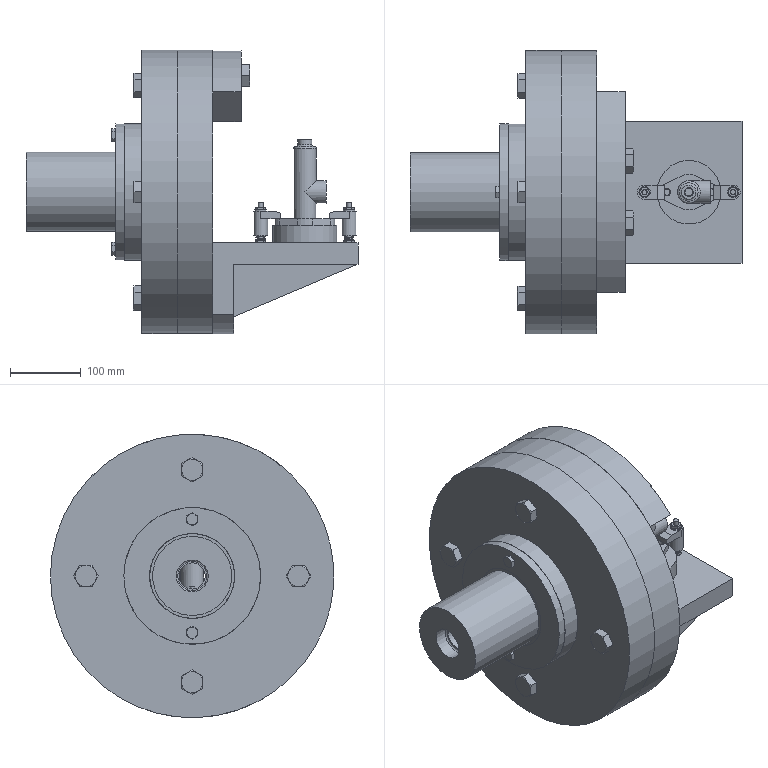Assembly | NX | mm | 33 component files | 33 solids | 523 faces | box 468.52 x 400 x 400 mm | volume 16620251 mm3 | plane 239 | cone 149 | cylinder 110 | torus 15 | spline 10 | commonest cylinder face diameters 19.623 x12 10 x10 6.985 x8 23 x8 27.7 x6 20 x5 9 x4 9.732 x4
Bill of materials:
unnamed part 1 | 1 |  | Solid stepped cylindrical pin: a short large-diameter head and a smaller coaxial shank, with chamfered edges.
unnamed part 2 | 1 |  | Tee-shaped tubular body. A vertical tube has a smaller stepped spigot at the top. A shorter side branch joins it at right angles. A thin two-lobed flange with two holes sits near the bottom, and the tube continues a short way below the flange.
unnamed part 3 | 1 |  | Stepped cylindrical pin with a thin round collar. Above the collar is a head with two parallel flats. Below it are a short undercut neck and a cylindrical shank with chamfered ends.
unnamed part 4 | 1 |  | Flanged bushing. A long cylindrical body leads to a short step, then a large round flange, then a short tapered nose. A central through bore has a counterbore or recessed ring on the flange face, and the flange has two small holes.
unnamed part 5 | 1 |  | Flat arc-shaped plate (annular sector) with radial-cut ends. One arc-shaped slot with rounded ends runs through it, concentric with the plate.
GB-T5782-2000,M20x80 | 6 |  | Hexagon Head Bolt, GB-T 5782-2000,M20x80
GB-T6172_1-2000,M8x1.25 | 4 |  | Hexagon Thin Nut, Chamfered, GB-T 6172.1-2000,M8x1.25
unnamed part 6 | 1 |  | Thick round disc with a central through hole and four small through holes equally spaced on a circle.
unnamed part 7 | 1 |  | Thin flat ring with a large central opening and two small through holes on opposite sides.
GB-T5783-2000,M10x30 | 2 |  | Hex-head bolt-like part: a hexagonal head with chamfered corners, a thin round washer face or collar under the head, and a smooth plain cylindrical shank with a chamfered flat end.
GB-T95-2002,M8 | 2 |  | Plain Washer, GB-T 95-2002,M8
unnamed part 8 | 2 |  | Solid cylinder with a flat lug on top. The lug has one rounded end, which holds a circular hole above the cylinder, and extends sideways to a rectangular end with a sloped top face.
unnamed part 9 | 2 |  | Helical coil spring of round wire with a constant diameter and roughly constant pitch. The end coils look closed and flattened.
GB-T70.1-2000,M12x40 | 2 |  | Hexagon Socket Head Cap Screw, GB-T 70.1-2000,M12x40
GB-T119.1-2000,10x50 | 2 |  | Parallel Pin, GB-T 119.1-2000,10x50
unnamed part 10 | 2 |  | Plain solid cylindrical rod or pin with flat ends.
unnamed part 11 | 1 |  | Thick round disc with a central through hole. It has four holes equally spaced on a circle, a group of three holes near one edge, and a group of five holes near the opposite edge (one larger hole with four smaller holes around it).
unnamed part 12 | 1 |  | Bracket block with a flat rectangular face and a cylindrical boss with a central bore. The block has a wedge-shaped (tapered) side profile with a small square foot at one end. Several small holes are visible, and the views also show four through holes, two slot-like features and a curved edge.
Mates:
1. concentric | adapter_plate 1 edge | faceplate 1 edge
2. concentric | CA614_spindle 1 edge | adapter_plate 1 edge
3. concentric | locking_plate 1 edge | CA614_spindle 1 edge
4. concentric | balance_block 1 edge | faceplate 1 edge
5. concentric | angle_iron 1 edge | faceplate 1 edge
6. concentric | cylinder_body 1 edge | angle_iron 1 edge
7. concentric | B_loc_pin 1 edge | angle_iron 1 edge
8. concentric | fixed_dowel_pin 1 edge | angle_iron 1 edge
9. distance | hook_clamp_plate 2 face | angle_iron 1 face
10. touch align | screw_rod 2 face | hook_clamp_plate 2 face
11. touch align | hook_clamp_plate 2 face | angle_iron 1 face
12. distance | screw_rod 2 face | hook_clamp_plate 2 face
13. concentric | GB-T6172_1-2000_M8x1_25 4 edge | angle_iron 1 arc
14. concentric | spring 2 edge | GB-T6172_1-2000_M8x1_25 4 edge
15. concentric | GB-T95-2002_M8 2 edge | hook_clamp_plate 2 edge
16. concentric | GB-T6172_1-2000_M8x1_25 3 edge | GB-T95-2002_M8 2 edge
17. bond | angle_iron 1 component | assembly component
18. bond | hook_clamp_plate 2 component | assembly component
19. bond | screw_rod 2 component | assembly component
20. bond | GB-T6172_1-2000_M8x1_25 4 component | assembly component
21. bond | spring 2 component | assembly component
22. bond | GB-T6172_1-2000_M8x1_25 3 component | assembly component
23. bond | GB-T95-2002_M8 2 component | assembly component
24. bond | hook_clamp_plate 1 component | assembly component
25. bond | screw_rod 1 component | assembly component
26. bond | GB-T6172_1-2000_M8x1_25 2 component | assembly component
27. bond | spring 1 component | assembly component
28. bond | GB-T6172_1-2000_M8x1_25 1 component | assembly component
29. bond | GB-T95-2002_M8 1 component | assembly component
30. circular | assembly datumaxis | assembly cartesiancoordinatesystem | assembly cartesiancoordinatesystem
31. circular | assembly datumaxis | assembly cartesiancoordinatesystem | assembly cartesiancoordinatesystem
32. circular | assembly datumaxis | assembly cartesiancoordinatesystem | assembly cartesiancoordinatesystem
33. circular | assembly datumaxis | assembly cartesiancoordinatesystem | assembly cartesiancoordinatesystem
34. circular | assembly datumaxis | assembly cartesiancoordinatesystem | assembly cartesiancoordinatesystem
35. circular | assembly datumaxis | assembly cartesiancoordinatesystem | assembly cartesiancoordinatesystem
36. bond | locking_plate 1 component | assembly component
37. bond | GB-T5783-2000_M10x30 2 component | assembly component
38. bond | GB-T5783-2000_M10x30 1 component | assembly component
39. circular | assembly datumaxis | assembly cartesiancoordinatesystem | assembly cartesiancoordinatesystem
40. bond | adapter_plate 1 component | assembly component
41. bond | GB-T5782-2000_M20x80 6 component | assembly component
42. bond | GB-T5782-2000_M20x80 3 component | assembly component
43. bond | GB-T5782-2000_M20x80 2 component | assembly component
44. bond | GB-T5782-2000_M20x80 1 component | assembly component
45. circular | assembly datumaxis | assembly cartesiancoordinatesystem | assembly cartesiancoordinatesystem | assembly cartesiancoordinatesystem | assembly cartesiancoordinatesystem
46. touch align | GB-T5782-2000_M20x80 5 face | faceplate 1 face
47. touch align | GB-T5782-2000_M20x80 4 face | faceplate 1 face
48. touch align | GB-T5782-2000_M20x80 4 face | balance_block 1 face
49. touch align | GB-T5782-2000_M20x80 5 face | balance_block 1 face